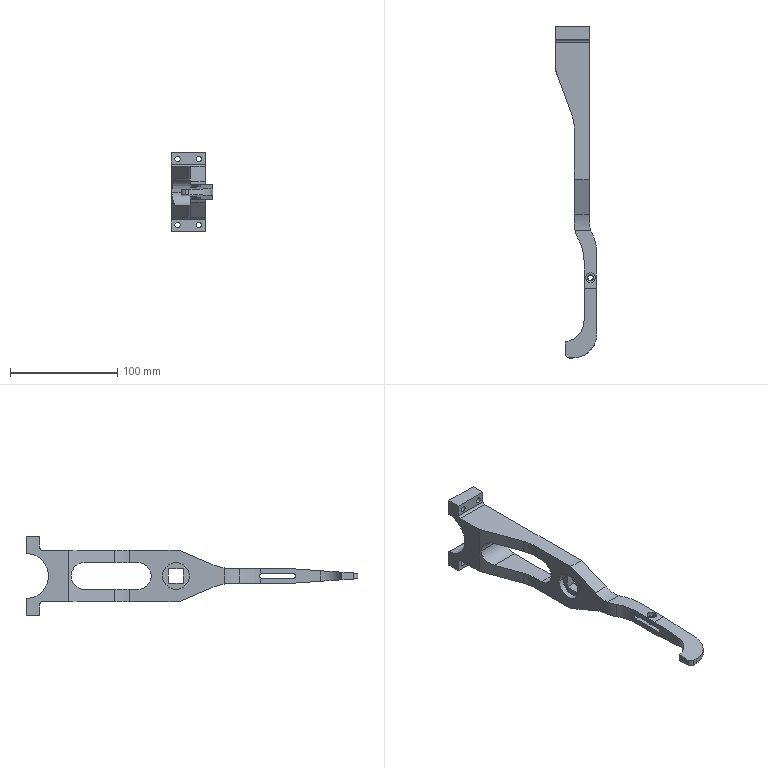Component | SolidWorks | AxleSupport-1 | 1 solid | 72 faces | volume 137963 mm3 | cylinder 38 | plane 32 | cone 2 | commonest cylinder face diameters 5 x12 80 x6 25 x5 4 x5 9 x2 60 x2 2 x2 40 x1